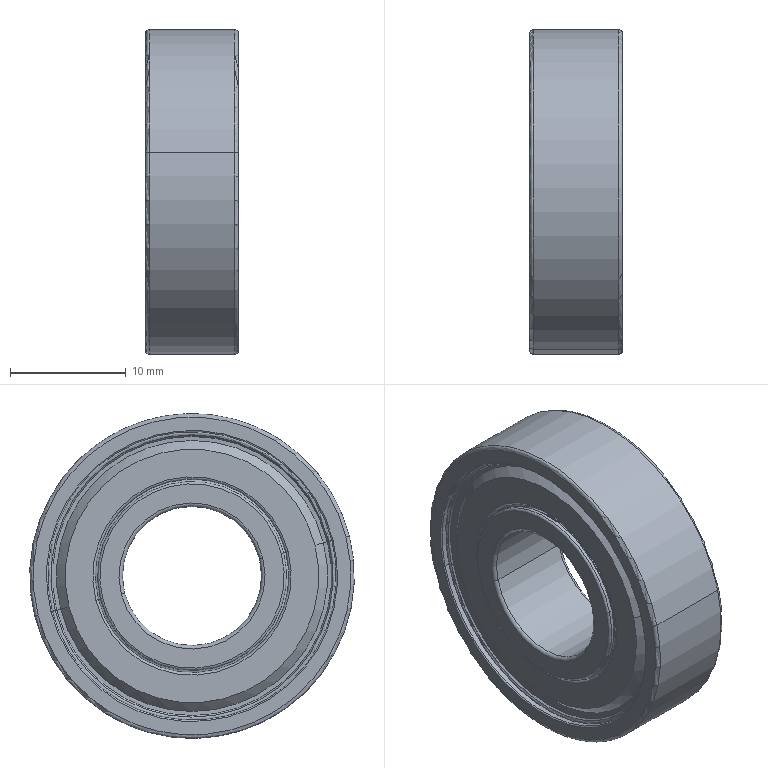Component | SolidWorks | BAU6001Z-1 | 1 solid | 80 faces | volume 3263 mm3 | torus 30 | cone 24 | cylinder 18 | plane 8 | commonest cylinder face diameters 17.5 x4 12 x2 16.3 x2 15.5 x2 17.1 x2 16.7 x2 24.9 x2 28 x2